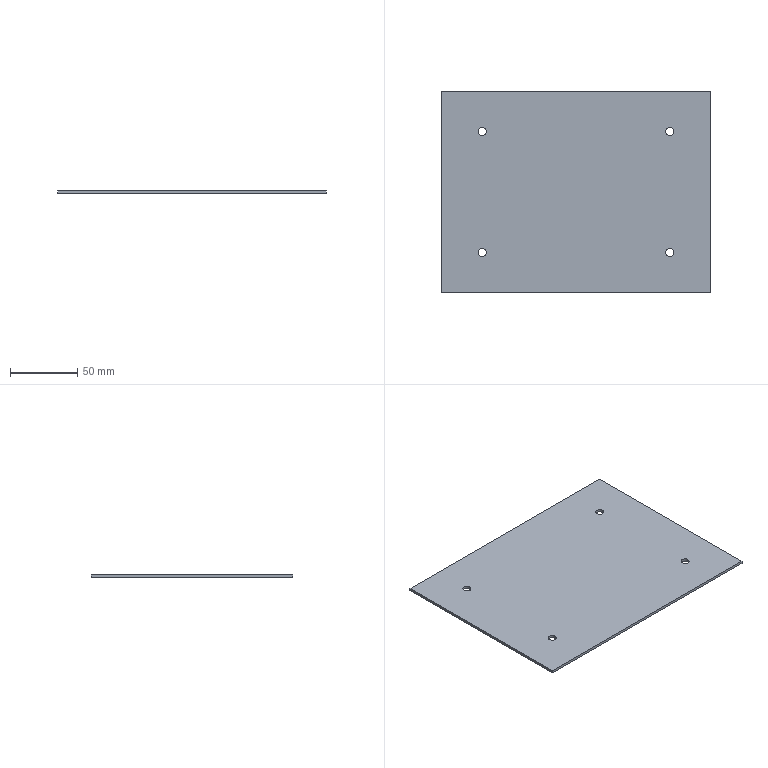Component | SolidWorks | RearFixingPlate-1 | 1 solid | 14 faces | box 200 x 150 x 2 mm | volume 59774 mm3 | cylinder 8 | plane 6 | commonest cylinder face diameters 6 x8
build123d program:
from build123d import *

# Parameters (mm, degrees)
SKETCH1_W           = 200
SKETCH1_H           = 150
SKETCH1_R           = 3
BOSS_EXTRUDE1_DEPTH = 2


with BuildPart() as part:
    # Sketch1 → Boss-Extrude1 (new body)
    with BuildSketch(Plane.XY):
        with Locations((29.76, 37.801)):
            Rectangle(SKETCH1_W, SKETCH1_H)
        with Locations((-40.24, 82.801)):
            Circle(SKETCH1_R, mode=Mode.SUBTRACT)
        with Locations((99.76, 82.801)):
            Circle(SKETCH1_R, mode=Mode.SUBTRACT)
        with Locations((-40.24, -7.199)):
            Circle(SKETCH1_R, mode=Mode.SUBTRACT)
        with Locations((99.76, -7.199)):
            Circle(SKETCH1_R, mode=Mode.SUBTRACT)
    extrude(amount=BOSS_EXTRUDE1_DEPTH)


solid = part.part

# Placed as in the assembly
solid = solid.moved(Location((218.065, 400.589, -395.236), (0, 0, 0)))
STEP:
#1=COLOUR_RGB('',0.7922,0.8196,0.9333);
#2=FILL_AREA_STYLE_COLOUR('',#1);
#3=FILL_AREA_STYLE('',(#2));
#4=SURFACE_STYLE_FILL_AREA(#3);
#5=SURFACE_SIDE_STYLE('',(#4));
#6=SURFACE_STYLE_USAGE(.BOTH.,#5);
#7=PRESENTATION_STYLE_ASSIGNMENT((#6));
#8=CARTESIAN_POINT('',(12.395,15.488,-15.482));
#9=VERTEX_POINT('',#8);
#10=CARTESIAN_POINT('',(12.631,15.488,-15.482));
#11=VERTEX_POINT('',#10);
#12=CARTESIAN_POINT('',(12.513,15.488,-15.482));
#13=DIRECTION('',(0.,0.,1.));
#14=DIRECTION('',(1.,0.,0.));
#15=AXIS2_PLACEMENT_3D('',#12,#13,#14);
#16=CIRCLE('',#15,0.1181);
#17=EDGE_CURVE('',#9,#11,#16,.T.);
#18=ORIENTED_EDGE('',*,*,#17,.T.);
#19=CARTESIAN_POINT('',(12.631,15.488,-15.56));
#20=VERTEX_POINT('',#19);
#21=CARTESIAN_POINT('',(12.631,15.488,-15.482));
#22=DIRECTION('',(0.,0.,-1.));
#23=VECTOR('',#22,39.37);
#24=LINE('',#21,#23);
#25=EDGE_CURVE('',#11,#20,#24,.T.);
#26=ORIENTED_EDGE('',*,*,#25,.T.);
#27=CARTESIAN_POINT('',(12.395,15.488,-15.56));
#28=VERTEX_POINT('',#27);
#29=CARTESIAN_POINT('',(12.513,15.488,-15.56));
#30=DIRECTION('',(0.,0.,1.));
#31=DIRECTION('',(1.,0.,0.));
#32=AXIS2_PLACEMENT_3D('',#29,#30,#31);
#33=CIRCLE('',#32,0.1181);
#34=EDGE_CURVE('',#28,#20,#33,.T.);
#35=ORIENTED_EDGE('',*,*,#34,.F.);
#36=CARTESIAN_POINT('',(12.395,15.488,-15.482));
#37=DIRECTION('',(0.,0.,-1.));
#38=VECTOR('',#37,39.37);
#39=LINE('',#36,#38);
#40=EDGE_CURVE('',#9,#28,#39,.T.);
#41=ORIENTED_EDGE('',*,*,#40,.F.);
#42=EDGE_LOOP('',(#18,#26,#35,#41));
#43=FACE_OUTER_BOUND('',#42,.T.);
#44=CARTESIAN_POINT('',(12.513,15.488,-15.482));
#45=DIRECTION('',(0.,0.,-1.));
#46=DIRECTION('',(-1.,0.,0.));
#47=AXIS2_PLACEMENT_3D('',#44,#45,#46);
#48=CYLINDRICAL_SURFACE('',#47,0.1181);
#49=ADVANCED_FACE('',(#43),#48,.F.);
#50=CARTESIAN_POINT('',(6.883,15.488,-15.482));
#51=VERTEX_POINT('',#50);
#52=CARTESIAN_POINT('',(7.119,15.488,-15.482));
#53=VERTEX_POINT('',#52);
#54=CARTESIAN_POINT('',(7.001,15.488,-15.482));
#55=DIRECTION('',(0.,0.,1.));
#56=DIRECTION('',(1.,0.,0.));
#57=AXIS2_PLACEMENT_3D('',#54,#55,#56);
#58=CIRCLE('',#57,0.1181);
#59=EDGE_CURVE('',#51,#53,#58,.T.);
#60=ORIENTED_EDGE('',*,*,#59,.T.);
#61=CARTESIAN_POINT('',(7.119,15.488,-15.56));
#62=VERTEX_POINT('',#61);
#63=CARTESIAN_POINT('',(7.119,15.488,-15.482));
#64=DIRECTION('',(0.,0.,-1.));
#65=VECTOR('',#64,39.37);
#66=LINE('',#63,#65);
#67=EDGE_CURVE('',#53,#62,#66,.T.);
#68=ORIENTED_EDGE('',*,*,#67,.T.);
#69=CARTESIAN_POINT('',(6.883,15.488,-15.56));
#70=VERTEX_POINT('',#69);
#71=CARTESIAN_POINT('',(7.001,15.488,-15.56));
#72=DIRECTION('',(0.,0.,1.));
#73=DIRECTION('',(1.,0.,0.));
#74=AXIS2_PLACEMENT_3D('',#71,#72,#73);
#75=CIRCLE('',#74,0.1181);
#76=EDGE_CURVE('',#70,#62,#75,.T.);
#77=ORIENTED_EDGE('',*,*,#76,.F.);
#78=CARTESIAN_POINT('',(6.883,15.488,-15.482));
#79=DIRECTION('',(0.,0.,-1.));
#80=VECTOR('',#79,39.37);
#81=LINE('',#78,#80);
#82=EDGE_CURVE('',#51,#70,#81,.T.);
#83=ORIENTED_EDGE('',*,*,#82,.F.);
#84=EDGE_LOOP('',(#60,#68,#77,#83));
#85=FACE_OUTER_BOUND('',#84,.T.);
#86=CARTESIAN_POINT('',(7.001,15.488,-15.482));
#87=DIRECTION('',(0.,0.,-1.));
#88=DIRECTION('',(-1.,0.,0.));
#89=AXIS2_PLACEMENT_3D('',#86,#87,#88);
#90=CYLINDRICAL_SURFACE('',#89,0.1181);
#91=ADVANCED_FACE('',(#85),#90,.F.);
#92=CARTESIAN_POINT('',(12.395,19.031,-15.482));
#93=VERTEX_POINT('',#92);
#94=CARTESIAN_POINT('',(12.631,19.031,-15.482));
#95=VERTEX_POINT('',#94);
#96=CARTESIAN_POINT('',(12.513,19.031,-15.482));
#97=DIRECTION('',(0.,0.,1.));
#98=DIRECTION('',(1.,0.,0.));
#99=AXIS2_PLACEMENT_3D('',#96,#97,#98);
#100=CIRCLE('',#99,0.1181);
#101=EDGE_CURVE('',#93,#95,#100,.T.);
#102=ORIENTED_EDGE('',*,*,#101,.T.);
#103=CARTESIAN_POINT('',(12.631,19.031,-15.56));
#104=VERTEX_POINT('',#103);
#105=CARTESIAN_POINT('',(12.631,19.031,-15.482));
#106=DIRECTION('',(0.,0.,-1.));
#107=VECTOR('',#106,39.37);
#108=LINE('',#105,#107);
#109=EDGE_CURVE('',#95,#104,#108,.T.);
#110=ORIENTED_EDGE('',*,*,#109,.T.);
#111=CARTESIAN_POINT('',(12.395,19.031,-15.56));
#112=VERTEX_POINT('',#111);
#113=CARTESIAN_POINT('',(12.513,19.031,-15.56));
#114=DIRECTION('',(0.,0.,1.));
#115=DIRECTION('',(1.,0.,0.));
#116=AXIS2_PLACEMENT_3D('',#113,#114,#115);
#117=CIRCLE('',#116,0.1181);
#118=EDGE_CURVE('',#112,#104,#117,.T.);
#119=ORIENTED_EDGE('',*,*,#118,.F.);
#120=CARTESIAN_POINT('',(12.395,19.031,-15.482));
#121=DIRECTION('',(0.,0.,-1.));
#122=VECTOR('',#121,39.37);
#123=LINE('',#120,#122);
#124=EDGE_CURVE('',#93,#112,#123,.T.);
#125=ORIENTED_EDGE('',*,*,#124,.F.);
#126=EDGE_LOOP('',(#102,#110,#119,#125));
#127=FACE_OUTER_BOUND('',#126,.T.);
#128=CARTESIAN_POINT('',(12.513,19.031,-15.482));
#129=DIRECTION('',(0.,0.,-1.));
#130=DIRECTION('',(-1.,0.,0.));
#131=AXIS2_PLACEMENT_3D('',#128,#129,#130);
#132=CYLINDRICAL_SURFACE('',#131,0.1181);
#133=ADVANCED_FACE('',(#127),#132,.F.);
#134=CARTESIAN_POINT('',(6.883,19.031,-15.482));
#135=VERTEX_POINT('',#134);
#136=CARTESIAN_POINT('',(7.119,19.031,-15.482));
#137=VERTEX_POINT('',#136);
#138=CARTESIAN_POINT('',(7.001,19.031,-15.482));
#139=DIRECTION('',(0.,0.,1.));
#140=DIRECTION('',(1.,0.,0.));
#141=AXIS2_PLACEMENT_3D('',#138,#139,#140);
#142=CIRCLE('',#141,0.1181);
#143=EDGE_CURVE('',#135,#137,#142,.T.);
#144=ORIENTED_EDGE('',*,*,#143,.T.);
#145=CARTESIAN_POINT('',(7.119,19.031,-15.56));
#146=VERTEX_POINT('',#145);
#147=CARTESIAN_POINT('',(7.119,19.031,-15.482));
#148=DIRECTION('',(0.,0.,-1.));
#149=VECTOR('',#148,39.37);
#150=LINE('',#147,#149);
#151=EDGE_CURVE('',#137,#146,#150,.T.);
#152=ORIENTED_EDGE('',*,*,#151,.T.);
#153=CARTESIAN_POINT('',(6.883,19.031,-15.56));
#154=VERTEX_POINT('',#153);
#155=CARTESIAN_POINT('',(7.001,19.031,-15.56));
#156=DIRECTION('',(0.,0.,1.));
#157=DIRECTION('',(1.,0.,0.));
#158=AXIS2_PLACEMENT_3D('',#155,#156,#157);
#159=CIRCLE('',#158,0.1181);
#160=EDGE_CURVE('',#154,#146,#159,.T.);
#161=ORIENTED_EDGE('',*,*,#160,.F.);
#162=CARTESIAN_POINT('',(6.883,19.031,-15.482));
#163=DIRECTION('',(0.,0.,-1.));
#164=VECTOR('',#163,39.37);
#165=LINE('',#162,#164);
#166=EDGE_CURVE('',#135,#154,#165,.T.);
#167=ORIENTED_EDGE('',*,*,#166,.F.);
#168=EDGE_LOOP('',(#144,#152,#161,#167));
#169=FACE_OUTER_BOUND('',#168,.T.);
#170=CARTESIAN_POINT('',(7.001,19.031,-15.482));
#171=DIRECTION('',(0.,0.,-1.));
#172=DIRECTION('',(-1.,0.,0.));
#173=AXIS2_PLACEMENT_3D('',#170,#171,#172);
#174=CYLINDRICAL_SURFACE('',#173,0.1181);
#175=ADVANCED_FACE('',(#169),#174,.F.);
#176=ORIENTED_EDGE('',*,*,#59,.F.);
#177=CARTESIAN_POINT('',(7.001,15.488,-15.482));
#178=DIRECTION('',(0.,0.,1.));
#179=DIRECTION('',(1.,0.,0.));
#180=AXIS2_PLACEMENT_3D('',#177,#178,#179);
#181=CIRCLE('',#180,0.1181);
#182=EDGE_CURVE('',#53,#51,#181,.T.);
#183=ORIENTED_EDGE('',*,*,#182,.F.);
#184=EDGE_LOOP('',(#176,#183));
#185=FACE_BOUND('',#184,.T.);
#186=ORIENTED_EDGE('',*,*,#143,.F.);
#187=CARTESIAN_POINT('',(7.001,19.031,-15.482));
#188=DIRECTION('',(0.,0.,1.));
#189=DIRECTION('',(1.,0.,0.));
#190=AXIS2_PLACEMENT_3D('',#187,#188,#189);
#191=CIRCLE('',#190,0.1181);
#192=EDGE_CURVE('',#137,#135,#191,.T.);
#193=ORIENTED_EDGE('',*,*,#192,.F.);
#194=EDGE_LOOP('',(#186,#193));
#195=FACE_BOUND('',#194,.T.);
#196=CARTESIAN_POINT('',(5.82,20.212,-15.482));
#197=VERTEX_POINT('',#196);
#198=CARTESIAN_POINT('',(5.82,14.307,-15.482));
#199=VERTEX_POINT('',#198);
#200=CARTESIAN_POINT('',(5.82,20.212,-15.482));
#201=DIRECTION('',(0.,-1.,0.));
#202=VECTOR('',#201,39.37);
#203=LINE('',#200,#202);
#204=EDGE_CURVE('',#197,#199,#203,.T.);
#205=ORIENTED_EDGE('',*,*,#204,.T.);
#206=CARTESIAN_POINT('',(13.694,14.307,-15.482));
#207=VERTEX_POINT('',#206);
#208=CARTESIAN_POINT('',(5.82,14.307,-15.482));
#209=DIRECTION('',(1.,0.,0.));
#210=VECTOR('',#209,39.37);
#211=LINE('',#208,#210);
#212=EDGE_CURVE('',#199,#207,#211,.T.);
#213=ORIENTED_EDGE('',*,*,#212,.T.);
#214=CARTESIAN_POINT('',(13.694,20.212,-15.482));
#215=VERTEX_POINT('',#214);
#216=CARTESIAN_POINT('',(13.694,20.212,-15.482));
#217=DIRECTION('',(0.,1.,0.));
#218=VECTOR('',#217,39.37);
#219=LINE('',#216,#218);
#220=EDGE_CURVE('',#207,#215,#219,.T.);
#221=ORIENTED_EDGE('',*,*,#220,.T.);
#222=CARTESIAN_POINT('',(5.82,20.212,-15.482));
#223=DIRECTION('',(-1.,-0.,0.));
#224=VECTOR('',#223,39.37);
#225=LINE('',#222,#224);
#226=EDGE_CURVE('',#215,#197,#225,.T.);
#227=ORIENTED_EDGE('',*,*,#226,.T.);
#228=EDGE_LOOP('',(#205,#213,#221,#227));
#229=FACE_OUTER_BOUND('',#228,.T.);
#230=ORIENTED_EDGE('',*,*,#101,.F.);
#231=CARTESIAN_POINT('',(12.513,19.031,-15.482));
#232=DIRECTION('',(0.,0.,1.));
#233=DIRECTION('',(1.,0.,0.));
#234=AXIS2_PLACEMENT_3D('',#231,#232,#233);
#235=CIRCLE('',#234,0.1181);
#236=EDGE_CURVE('',#95,#93,#235,.T.);
#237=ORIENTED_EDGE('',*,*,#236,.F.);
#238=EDGE_LOOP('',(#230,#237));
#239=FACE_BOUND('',#238,.T.);
#240=ORIENTED_EDGE('',*,*,#17,.F.);
#241=CARTESIAN_POINT('',(12.513,15.488,-15.482));
#242=DIRECTION('',(0.,0.,1.));
#243=DIRECTION('',(1.,0.,0.));
#244=AXIS2_PLACEMENT_3D('',#241,#242,#243);
#245=CIRCLE('',#244,0.1181);
#246=EDGE_CURVE('',#11,#9,#245,.T.);
#247=ORIENTED_EDGE('',*,*,#246,.F.);
#248=EDGE_LOOP('',(#240,#247));
#249=FACE_BOUND('',#248,.T.);
#250=CARTESIAN_POINT('',(8.585,15.771,-15.482));
#251=DIRECTION('',(0.,0.,1.));
#252=DIRECTION('',(1.,0.,0.));
#253=AXIS2_PLACEMENT_3D('',#250,#251,#252);
#254=PLANE('',#253);
#255=ADVANCED_FACE('',(#185,#195,#229,#239,#249),#254,.T.);
#256=CARTESIAN_POINT('',(5.82,20.212,-15.56));
#257=VERTEX_POINT('',#256);
#258=CARTESIAN_POINT('',(5.82,14.307,-15.56));
#259=VERTEX_POINT('',#258);
#260=CARTESIAN_POINT('',(5.82,20.212,-15.56));
#261=DIRECTION('',(0.,-1.,0.));
#262=VECTOR('',#261,39.37);
#263=LINE('',#260,#262);
#264=EDGE_CURVE('',#257,#259,#263,.T.);
#265=ORIENTED_EDGE('',*,*,#264,.F.);
#266=CARTESIAN_POINT('',(13.694,20.212,-15.56));
#267=VERTEX_POINT('',#266);
#268=CARTESIAN_POINT('',(5.82,20.212,-15.56));
#269=DIRECTION('',(-1.,-0.,0.));
#270=VECTOR('',#269,39.37);
#271=LINE('',#268,#270);
#272=EDGE_CURVE('',#267,#257,#271,.T.);
#273=ORIENTED_EDGE('',*,*,#272,.F.);
#274=CARTESIAN_POINT('',(13.694,14.307,-15.56));
#275=VERTEX_POINT('',#274);
#276=CARTESIAN_POINT('',(13.694,20.212,-15.56));
#277=DIRECTION('',(0.,1.,0.));
#278=VECTOR('',#277,39.37);
#279=LINE('',#276,#278);
#280=EDGE_CURVE('',#275,#267,#279,.T.);
#281=ORIENTED_EDGE('',*,*,#280,.F.);
#282=CARTESIAN_POINT('',(5.82,14.307,-15.56));
#283=DIRECTION('',(1.,0.,0.));
#284=VECTOR('',#283,39.37);
#285=LINE('',#282,#284);
#286=EDGE_CURVE('',#259,#275,#285,.T.);
#287=ORIENTED_EDGE('',*,*,#286,.F.);
#288=EDGE_LOOP('',(#265,#273,#281,#287));
#289=FACE_OUTER_BOUND('',#288,.T.);
#290=ORIENTED_EDGE('',*,*,#160,.T.);
#291=CARTESIAN_POINT('',(7.001,19.031,-15.56));
#292=DIRECTION('',(0.,0.,1.));
#293=DIRECTION('',(1.,0.,0.));
#294=AXIS2_PLACEMENT_3D('',#291,#292,#293);
#295=CIRCLE('',#294,0.1181);
#296=EDGE_CURVE('',#146,#154,#295,.T.);
#297=ORIENTED_EDGE('',*,*,#296,.T.);
#298=EDGE_LOOP('',(#290,#297));
#299=FACE_BOUND('',#298,.T.);
#300=ORIENTED_EDGE('',*,*,#118,.T.);
#301=CARTESIAN_POINT('',(12.513,19.031,-15.56));
#302=DIRECTION('',(0.,0.,1.));
#303=DIRECTION('',(1.,0.,0.));
#304=AXIS2_PLACEMENT_3D('',#301,#302,#303);
#305=CIRCLE('',#304,0.1181);
#306=EDGE_CURVE('',#104,#112,#305,.T.);
#307=ORIENTED_EDGE('',*,*,#306,.T.);
#308=EDGE_LOOP('',(#300,#307));
#309=FACE_BOUND('',#308,.T.);
#310=ORIENTED_EDGE('',*,*,#76,.T.);
#311=CARTESIAN_POINT('',(7.001,15.488,-15.56));
#312=DIRECTION('',(0.,0.,1.));
#313=DIRECTION('',(1.,0.,0.));
#314=AXIS2_PLACEMENT_3D('',#311,#312,#313);
#315=CIRCLE('',#314,0.1181);
#316=EDGE_CURVE('',#62,#70,#315,.T.);
#317=ORIENTED_EDGE('',*,*,#316,.T.);
#318=EDGE_LOOP('',(#310,#317));
#319=FACE_BOUND('',#318,.T.);
#320=ORIENTED_EDGE('',*,*,#34,.T.);
#321=CARTESIAN_POINT('',(12.513,15.488,-15.56));
#322=DIRECTION('',(0.,0.,1.));
#323=DIRECTION('',(1.,0.,0.));
#324=AXIS2_PLACEMENT_3D('',#321,#322,#323);
#325=CIRCLE('',#324,0.1181);
#326=EDGE_CURVE('',#20,#28,#325,.T.);
#327=ORIENTED_EDGE('',*,*,#326,.T.);
#328=EDGE_LOOP('',(#320,#327));
#329=FACE_BOUND('',#328,.T.);
#330=CARTESIAN_POINT('',(8.585,15.771,-15.56));
#331=DIRECTION('',(0.,0.,1.));
#332=DIRECTION('',(1.,0.,0.));
#333=AXIS2_PLACEMENT_3D('',#330,#331,#332);
#334=PLANE('',#333);
#335=ADVANCED_FACE('',(#289,#299,#309,#319,#329),#334,.F.);
#336=ORIENTED_EDGE('',*,*,#264,.T.);
#337=CARTESIAN_POINT('',(5.82,14.307,-15.482));
#338=DIRECTION('',(0.,0.,-1.));
#339=VECTOR('',#338,39.37);
#340=LINE('',#337,#339);
#341=EDGE_CURVE('',#199,#259,#340,.T.);
#342=ORIENTED_EDGE('',*,*,#341,.F.);
#343=ORIENTED_EDGE('',*,*,#204,.F.);
#344=CARTESIAN_POINT('',(5.82,20.212,-15.482));
#345=DIRECTION('',(0.,0.,-1.));
#346=VECTOR('',#345,39.37);
#347=LINE('',#344,#346);
#348=EDGE_CURVE('',#197,#257,#347,.T.);
#349=ORIENTED_EDGE('',*,*,#348,.T.);
#350=EDGE_LOOP('',(#336,#342,#343,#349));
#351=FACE_OUTER_BOUND('',#350,.T.);
#352=CARTESIAN_POINT('',(5.82,20.212,-15.482));
#353=DIRECTION('',(1.,0.,0.));
#354=DIRECTION('',(-0.,1.,0.));
#355=AXIS2_PLACEMENT_3D('',#352,#353,#354);
#356=PLANE('',#355);
#357=ADVANCED_FACE('',(#351),#356,.F.);
#358=ORIENTED_EDGE('',*,*,#286,.T.);
#359=CARTESIAN_POINT('',(13.694,14.307,-15.482));
#360=DIRECTION('',(0.,0.,-1.));
#361=VECTOR('',#360,39.37);
#362=LINE('',#359,#361);
#363=EDGE_CURVE('',#207,#275,#362,.T.);
#364=ORIENTED_EDGE('',*,*,#363,.F.);
#365=ORIENTED_EDGE('',*,*,#212,.F.);
#366=ORIENTED_EDGE('',*,*,#341,.T.);
#367=EDGE_LOOP('',(#358,#364,#365,#366));
#368=FACE_OUTER_BOUND('',#367,.T.);
#369=CARTESIAN_POINT('',(5.82,14.307,-15.482));
#370=DIRECTION('',(0.,1.,0.));
#371=DIRECTION('',(0.,0.,1.));
#372=AXIS2_PLACEMENT_3D('',#369,#370,#371);
#373=PLANE('',#372);
#374=ADVANCED_FACE('',(#368),#373,.F.);
#375=ORIENTED_EDGE('',*,*,#280,.T.);
#376=CARTESIAN_POINT('',(13.694,20.212,-15.482));
#377=DIRECTION('',(0.,0.,-1.));
#378=VECTOR('',#377,39.37);
#379=LINE('',#376,#378);
#380=EDGE_CURVE('',#215,#267,#379,.T.);
#381=ORIENTED_EDGE('',*,*,#380,.F.);
#382=ORIENTED_EDGE('',*,*,#220,.F.);
#383=ORIENTED_EDGE('',*,*,#363,.T.);
#384=EDGE_LOOP('',(#375,#381,#382,#383));
#385=FACE_OUTER_BOUND('',#384,.T.);
#386=CARTESIAN_POINT('',(13.694,20.212,-15.482));
#387=DIRECTION('',(-1.,0.,0.));
#388=DIRECTION('',(0.,0.,1.));
#389=AXIS2_PLACEMENT_3D('',#386,#387,#388);
#390=PLANE('',#389);
#391=ADVANCED_FACE('',(#385),#390,.F.);
#392=ORIENTED_EDGE('',*,*,#272,.T.);
#393=ORIENTED_EDGE('',*,*,#348,.F.);
#394=ORIENTED_EDGE('',*,*,#226,.F.);
#395=ORIENTED_EDGE('',*,*,#380,.T.);
#396=EDGE_LOOP('',(#392,#393,#394,#395));
#397=FACE_OUTER_BOUND('',#396,.T.);
#398=CARTESIAN_POINT('',(5.82,20.212,-15.482));
#399=DIRECTION('',(0.,-1.,0.));
#400=DIRECTION('',(1.,0.,0.));
#401=AXIS2_PLACEMENT_3D('',#398,#399,#400);
#402=PLANE('',#401);
#403=ADVANCED_FACE('',(#397),#402,.F.);
#404=ORIENTED_EDGE('',*,*,#151,.F.);
#405=ORIENTED_EDGE('',*,*,#192,.T.);
#406=ORIENTED_EDGE('',*,*,#166,.T.);
#407=ORIENTED_EDGE('',*,*,#296,.F.);
#408=EDGE_LOOP('',(#404,#405,#406,#407));
#409=FACE_OUTER_BOUND('',#408,.T.);
#410=CARTESIAN_POINT('',(7.001,19.031,-15.482));
#411=DIRECTION('',(0.,0.,-1.));
#412=DIRECTION('',(-1.,0.,0.));
#413=AXIS2_PLACEMENT_3D('',#410,#411,#412);
#414=CYLINDRICAL_SURFACE('',#413,0.1181);
#415=ADVANCED_FACE('',(#409),#414,.F.);
#416=ORIENTED_EDGE('',*,*,#109,.F.);
#417=ORIENTED_EDGE('',*,*,#236,.T.);
#418=ORIENTED_EDGE('',*,*,#124,.T.);
#419=ORIENTED_EDGE('',*,*,#306,.F.);
#420=EDGE_LOOP('',(#416,#417,#418,#419));
#421=FACE_OUTER_BOUND('',#420,.T.);
#422=CARTESIAN_POINT('',(12.513,19.031,-15.482));
#423=DIRECTION('',(0.,0.,-1.));
#424=DIRECTION('',(-1.,0.,0.));
#425=AXIS2_PLACEMENT_3D('',#422,#423,#424);
#426=CYLINDRICAL_SURFACE('',#425,0.1181);
#427=ADVANCED_FACE('',(#421),#426,.F.);
#428=ORIENTED_EDGE('',*,*,#67,.F.);
#429=ORIENTED_EDGE('',*,*,#182,.T.);
#430=ORIENTED_EDGE('',*,*,#82,.T.);
#431=ORIENTED_EDGE('',*,*,#316,.F.);
#432=EDGE_LOOP('',(#428,#429,#430,#431));
#433=FACE_OUTER_BOUND('',#432,.T.);
#434=CARTESIAN_POINT('',(7.001,15.488,-15.482));
#435=DIRECTION('',(0.,0.,-1.));
#436=DIRECTION('',(-1.,0.,0.));
#437=AXIS2_PLACEMENT_3D('',#434,#435,#436);
#438=CYLINDRICAL_SURFACE('',#437,0.1181);
#439=ADVANCED_FACE('',(#433),#438,.F.);
#440=ORIENTED_EDGE('',*,*,#25,.F.);
#441=ORIENTED_EDGE('',*,*,#246,.T.);
#442=ORIENTED_EDGE('',*,*,#40,.T.);
#443=ORIENTED_EDGE('',*,*,#326,.F.);
#444=EDGE_LOOP('',(#440,#441,#442,#443));
#445=FACE_OUTER_BOUND('',#444,.T.);
#446=CARTESIAN_POINT('',(12.513,15.488,-15.482));
#447=DIRECTION('',(0.,0.,-1.));
#448=DIRECTION('',(-1.,0.,0.));
#449=AXIS2_PLACEMENT_3D('',#446,#447,#448);
#450=CYLINDRICAL_SURFACE('',#449,0.1181);
#451=ADVANCED_FACE('',(#445),#450,.F.);
#452=CLOSED_SHELL('',(#49,#91,#133,#175,#255,#335,#357,#374,#391,#403,#415,#427,#439,#451));
#453=MANIFOLD_SOLID_BREP('',#452);
#454=STYLED_ITEM('',(#7),#453);
#455=PRESENTATION_LAYER_ASSIGNMENT('','',(#454));
#456=(LENGTH_UNIT()NAMED_UNIT(*)SI_UNIT($,.METRE.));
#457=LENGTH_MEASURE_WITH_UNIT(LENGTH_MEASURE(0.0254),#456);
#458=DIMENSIONAL_EXPONENTS(1.,0.,0.,0.,0.,0.,0.);
#459=(CONVERSION_BASED_UNIT('',#457)LENGTH_UNIT()NAMED_UNIT(#458));
#460=UNCERTAINTY_MEASURE_WITH_UNIT(LENGTH_MEASURE(0.00001),#459,'','');
#461=(NAMED_UNIT(*)PLANE_ANGLE_UNIT()SI_UNIT($,.RADIAN.));
#462=(NAMED_UNIT(*)SI_UNIT($,.STERADIAN.)SOLID_ANGLE_UNIT());
#463=(GEOMETRIC_REPRESENTATION_CONTEXT(3)GLOBAL_UNCERTAINTY_ASSIGNED_CONTEXT((#460))GLOBAL_UNIT_ASSIGNED_CONTEXT((#459,#461,#462))REPRESENTATION_CONTEXT('',''));
#464=MECHANICAL_DESIGN_GEOMETRIC_PRESENTATION_REPRESENTATION('',(#454),#463);
#465=CARTESIAN_POINT('',(0.,0.,0.));
#466=DIRECTION('',(0.,0.,1.));
#467=DIRECTION('',(1.,0.,0.));
#468=AXIS2_PLACEMENT_3D('',#465,#466,#467);
#469=(LENGTH_UNIT()NAMED_UNIT(*)SI_UNIT($,.METRE.));
#470=LENGTH_MEASURE_WITH_UNIT(LENGTH_MEASURE(0.0254),#469);
#471=DIMENSIONAL_EXPONENTS(1.,0.,0.,0.,0.,0.,0.);
#472=(CONVERSION_BASED_UNIT('',#470)LENGTH_UNIT()NAMED_UNIT(#471));
#473=UNCERTAINTY_MEASURE_WITH_UNIT(LENGTH_MEASURE(0.00001),#472,'','');
#474=(NAMED_UNIT(*)PLANE_ANGLE_UNIT()SI_UNIT($,.RADIAN.));
#475=(NAMED_UNIT(*)SI_UNIT($,.STERADIAN.)SOLID_ANGLE_UNIT());
#476=(GEOMETRIC_REPRESENTATION_CONTEXT(3)GLOBAL_UNCERTAINTY_ASSIGNED_CONTEXT((#473))GLOBAL_UNIT_ASSIGNED_CONTEXT((#472,#474,#475))REPRESENTATION_CONTEXT('',''));
#477=ADVANCED_BREP_SHAPE_REPRESENTATION('',(#453,#468),#476);